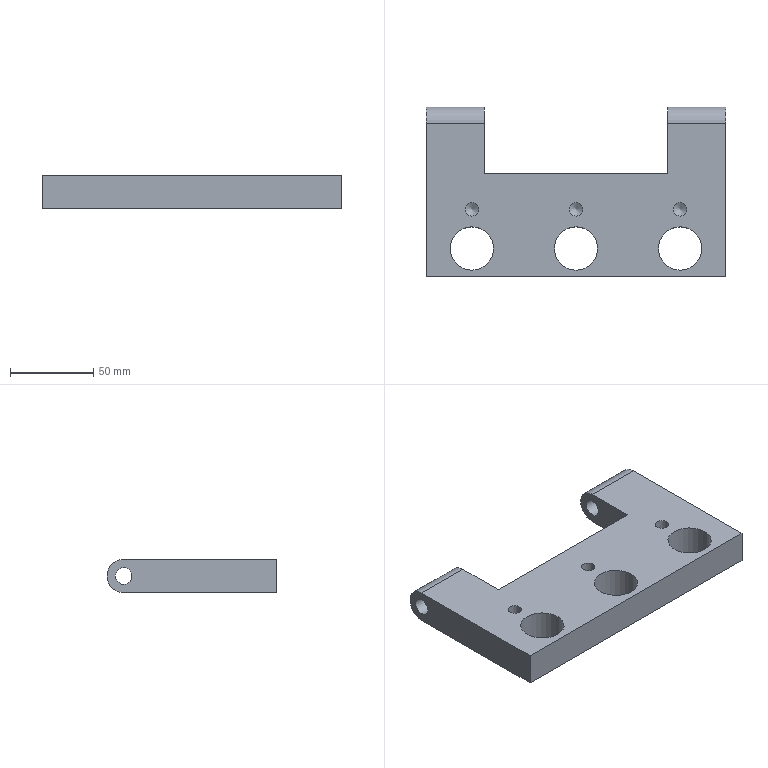Component | NX | DRILL_TEMPLATE | 1 solid | 21 faces | volume 236308 mm3 | cylinder 10 | plane 8 | cone 3 | commonest cylinder face diameters 26 x3 8 x3 20 x2 10 x2